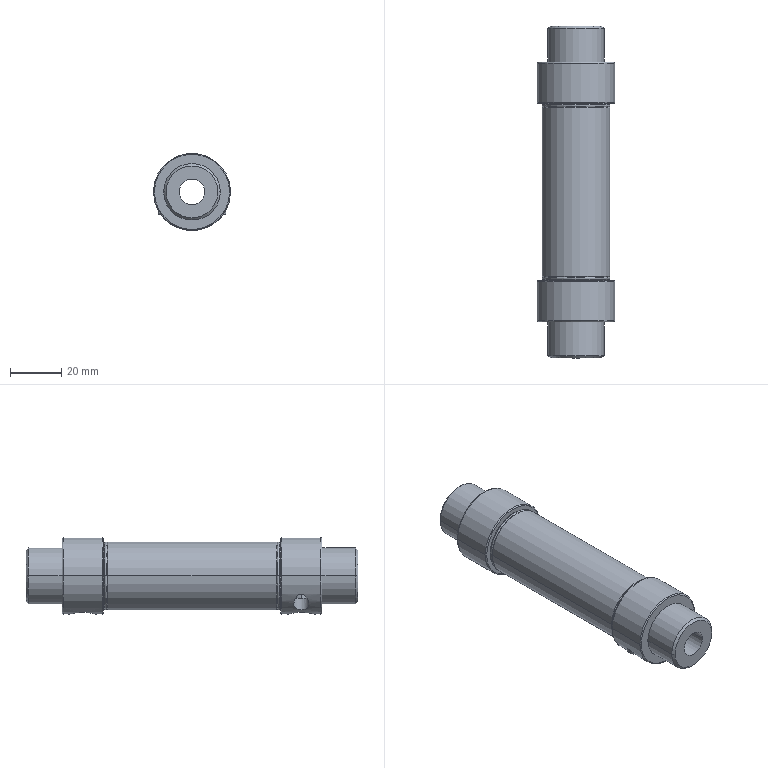Component | SolidWorks | MACJ25x25-10S-Body-1_MACJ25x25-10S-Body-1 | 1 solid | 66 faces | box 30 x 129 x 30 mm | volume 40132 mm3 | cylinder 26 | cone 16 | torus 12 | plane 12 | commonest cylinder face diameters 6 x6 10 x4 9.73 x4 22 x4 30 x4 25 x2 26.4 x2
build123d program:
from build123d import *

# Parameters (mm, degrees)
SKETCH6_W = 3
SKETCH6_H = 9
SKETCH7_W = 3
SKETCH7_H = 9
SKETCH8_W = 3
SKETCH8_H = 3.75
SKETCH9_W = 3
SKETCH9_H = 3.75


with BuildPart() as part:
    # Sketch1 → Revolve1 (revolve)
    with BuildSketch(Plane.XY, mode=Mode.PRIVATE) as revolve1_sk:
        with BuildLine():
            Line((0, 0), (0, 10.08))
            Line((0, 10.08), (0.92, 11))
            Line((0.92, 11), (14, 11))
            Line((14, 11), (14, 14.6))
            ThreePointArc((14, 14.6), (14.117, 14.883), (14.4, 15))
            Line((14.4, 15), (29.6, 15))
            ThreePointArc((29.6, 15), (29.883, 14.883), (30, 14.6))
            Line((30, 14.6), (30, 12.7))
            Line((30, 12.7), (30.62, 13.101))
            ThreePointArc((30.62, 13.101), (31.038, 13.196), (31.42, 13))
            Line((31.42, 13), (31.7, 13.2))
            Line((31.7, 13.2), (97.3, 13.2))
            Line((97.3, 13.2), (97.58, 13))
            ThreePointArc((97.58, 13), (97.962, 13.196), (98.38, 13.101))
            Line((98.38, 13.101), (99, 12.7))
            Line((99, 12.7), (99, 14.6))
            ThreePointArc((99, 14.6), (99.117, 14.883), (99.4, 15))
            Line((99.4, 15), (114.6, 15))
            ThreePointArc((114.6, 15), (114.883, 14.883), (115, 14.6))
            Line((115, 14.6), (115, 0))
            Line((115, 0), (0, 0))
        make_face()
    revolve(revolve1_sk.sketch.rotate(Axis((115, 0, 0), (-1, 0, 0)), 270), axis=Axis((115, 0, 0), (-1, 0, 0)))

    # Sketch2 → Revolve2 (revolve)
    with BuildSketch(Plane.XY, mode=Mode.PRIVATE) as revolve2_sk:
        Polygon((115, 0), (115, 11), (128.08, 11), (129, 10.08), (129, 0), align=None)
    revolve(revolve2_sk.sketch.rotate(Axis((129, 0, 0), (-1, 0, 0)), 270), axis=Axis((129, 0, 0), (-1, 0, 0)))

    # Sketch3 → Cut-Revolve1 (revolve, cut)
    with BuildSketch(Plane.XY, mode=Mode.PRIVATE) as cut_revolve1_sk:
        Polygon((22, 15), (27.446, 15), (26.865, 14.419), (26.865, 7), (22, 7), align=None)
    revolve(cut_revolve1_sk.sketch.rotate(Axis((22, 7, 0), (0, 1, 0)), 270), axis=Axis((22, 7, 0), (0, 1, 0)), mode=Mode.SUBTRACT)

    # Sketch4 → Cut-Revolve2 (revolve, cut)
    with BuildSketch(Plane.XY, mode=Mode.PRIVATE) as cut_revolve2_sk:
        Polygon((107, 15), (112.446, 15), (111.865, 14.419), (111.865, 7), (107, 7), align=None)
    revolve(cut_revolve2_sk.sketch.rotate(Axis((107, 7, 0), (0, 1, 0)), 270), axis=Axis((107, 7, 0), (0, 1, 0)), mode=Mode.SUBTRACT)

    # Sketch5 → Cut-Revolve3 (revolve, cut)
    with BuildSketch(Plane.XY, mode=Mode.PRIVATE) as cut_revolve3_sk:
        Polygon((0, 0), (0, 5), (41, 5), (41, 12.5), (88, 12.5), (88, 5), (129, 5), (129, 0), align=None)
    revolve(cut_revolve3_sk.sketch.rotate(Axis((129, 0, 0), (-1, 0, 0)), 270), axis=Axis((129, 0, 0), (-1, 0, 0)), mode=Mode.SUBTRACT)

    # Sketch6 → Cut-Revolve4 (revolve, cut)
    with BuildSketch(Plane.XY.offset(10.2), mode=Mode.PRIVATE) as cut_revolve4_sk:
        with Locations((23.5, 9.5)):
            Rectangle(SKETCH6_W, SKETCH6_H)
    revolve(cut_revolve4_sk.sketch.rotate(Axis((22, 5, 10.2), (0, 1, 0)), 270), axis=Axis((22, 5, 10.2), (0, 1, 0)), mode=Mode.SUBTRACT)

    # Sketch7 → Cut-Revolve5 (revolve, cut)
    with BuildSketch(Plane.XY.offset(-10.2)):
        with Locations((108.5, 12)):
            Rectangle(SKETCH7_W, SKETCH7_H)
    revolve(axis=Axis((107, 7.5, -10.2), (0, 1, 0)), mode=Mode.SUBTRACT)

    # Sketch8 → Revolve3 (revolve)
    with BuildSketch(Plane.XY.offset(10.2)):
        with Locations((23.5, 6.875)):
            Rectangle(SKETCH8_W, SKETCH8_H)
    revolve(axis=Axis((22, 5, 10.2), (0, 1, 0)))

    # Sketch9 → Revolve4 (revolve)
    with BuildSketch(Plane.XY.offset(-10.2)):
        with Locations((108.5, 6.875)):
            Rectangle(SKETCH9_W, SKETCH9_H)
    revolve(axis=Axis((107, 5, -10.2), (0, 1, 0)))


solid = part.part

# Placed as in the assembly
solid = solid.moved(Location((-4.335, 187.168, -163.015), (-90, 90, 0)))